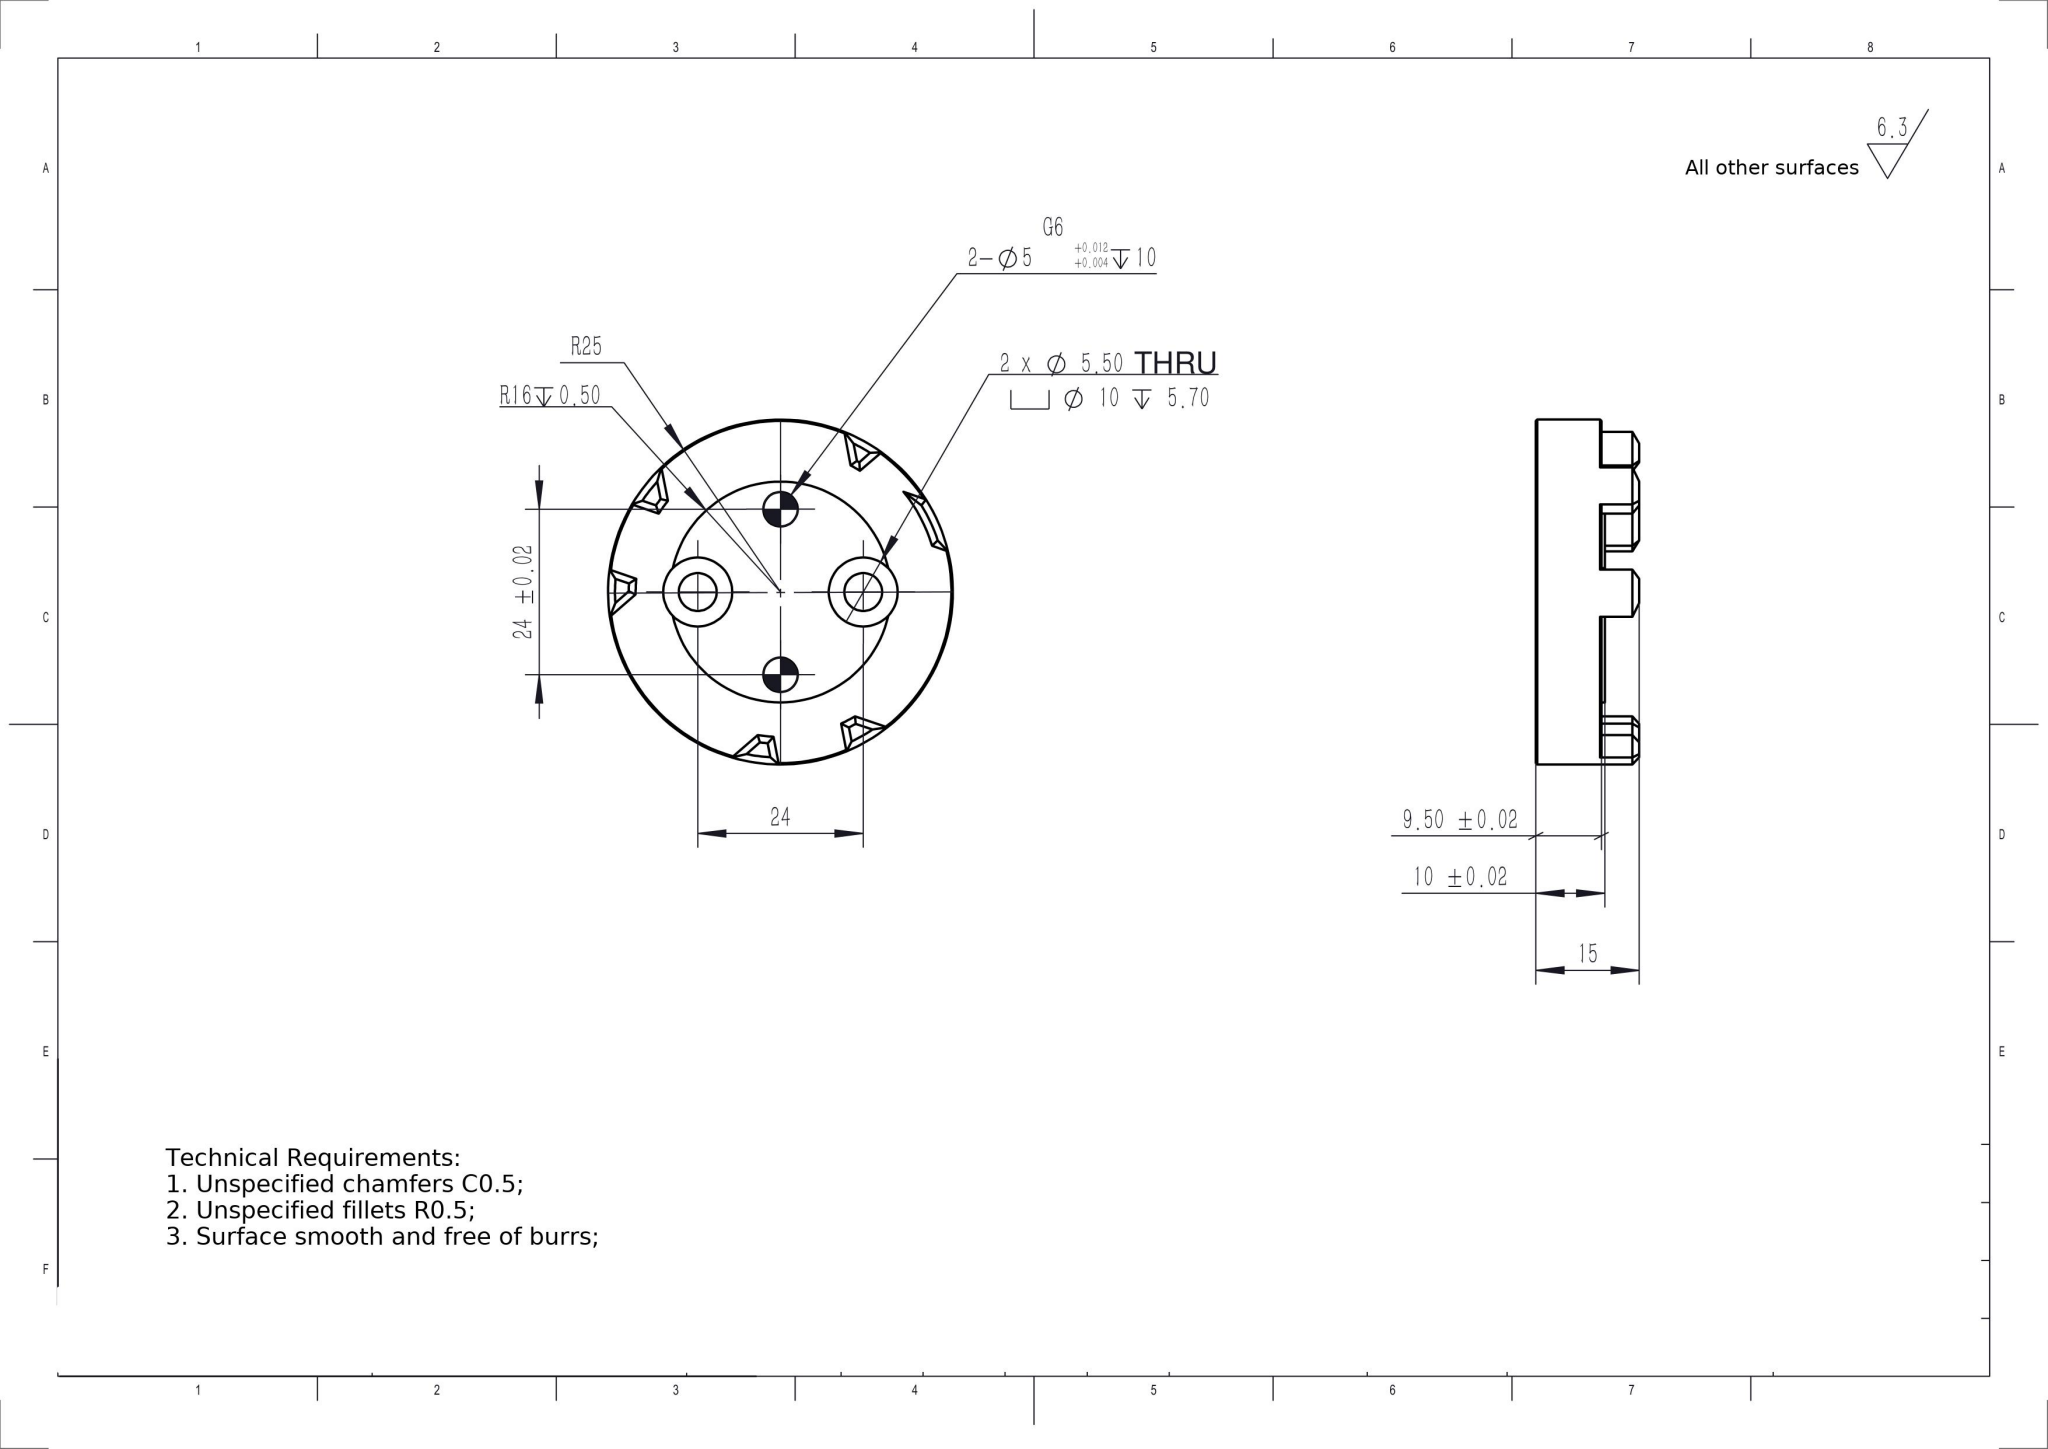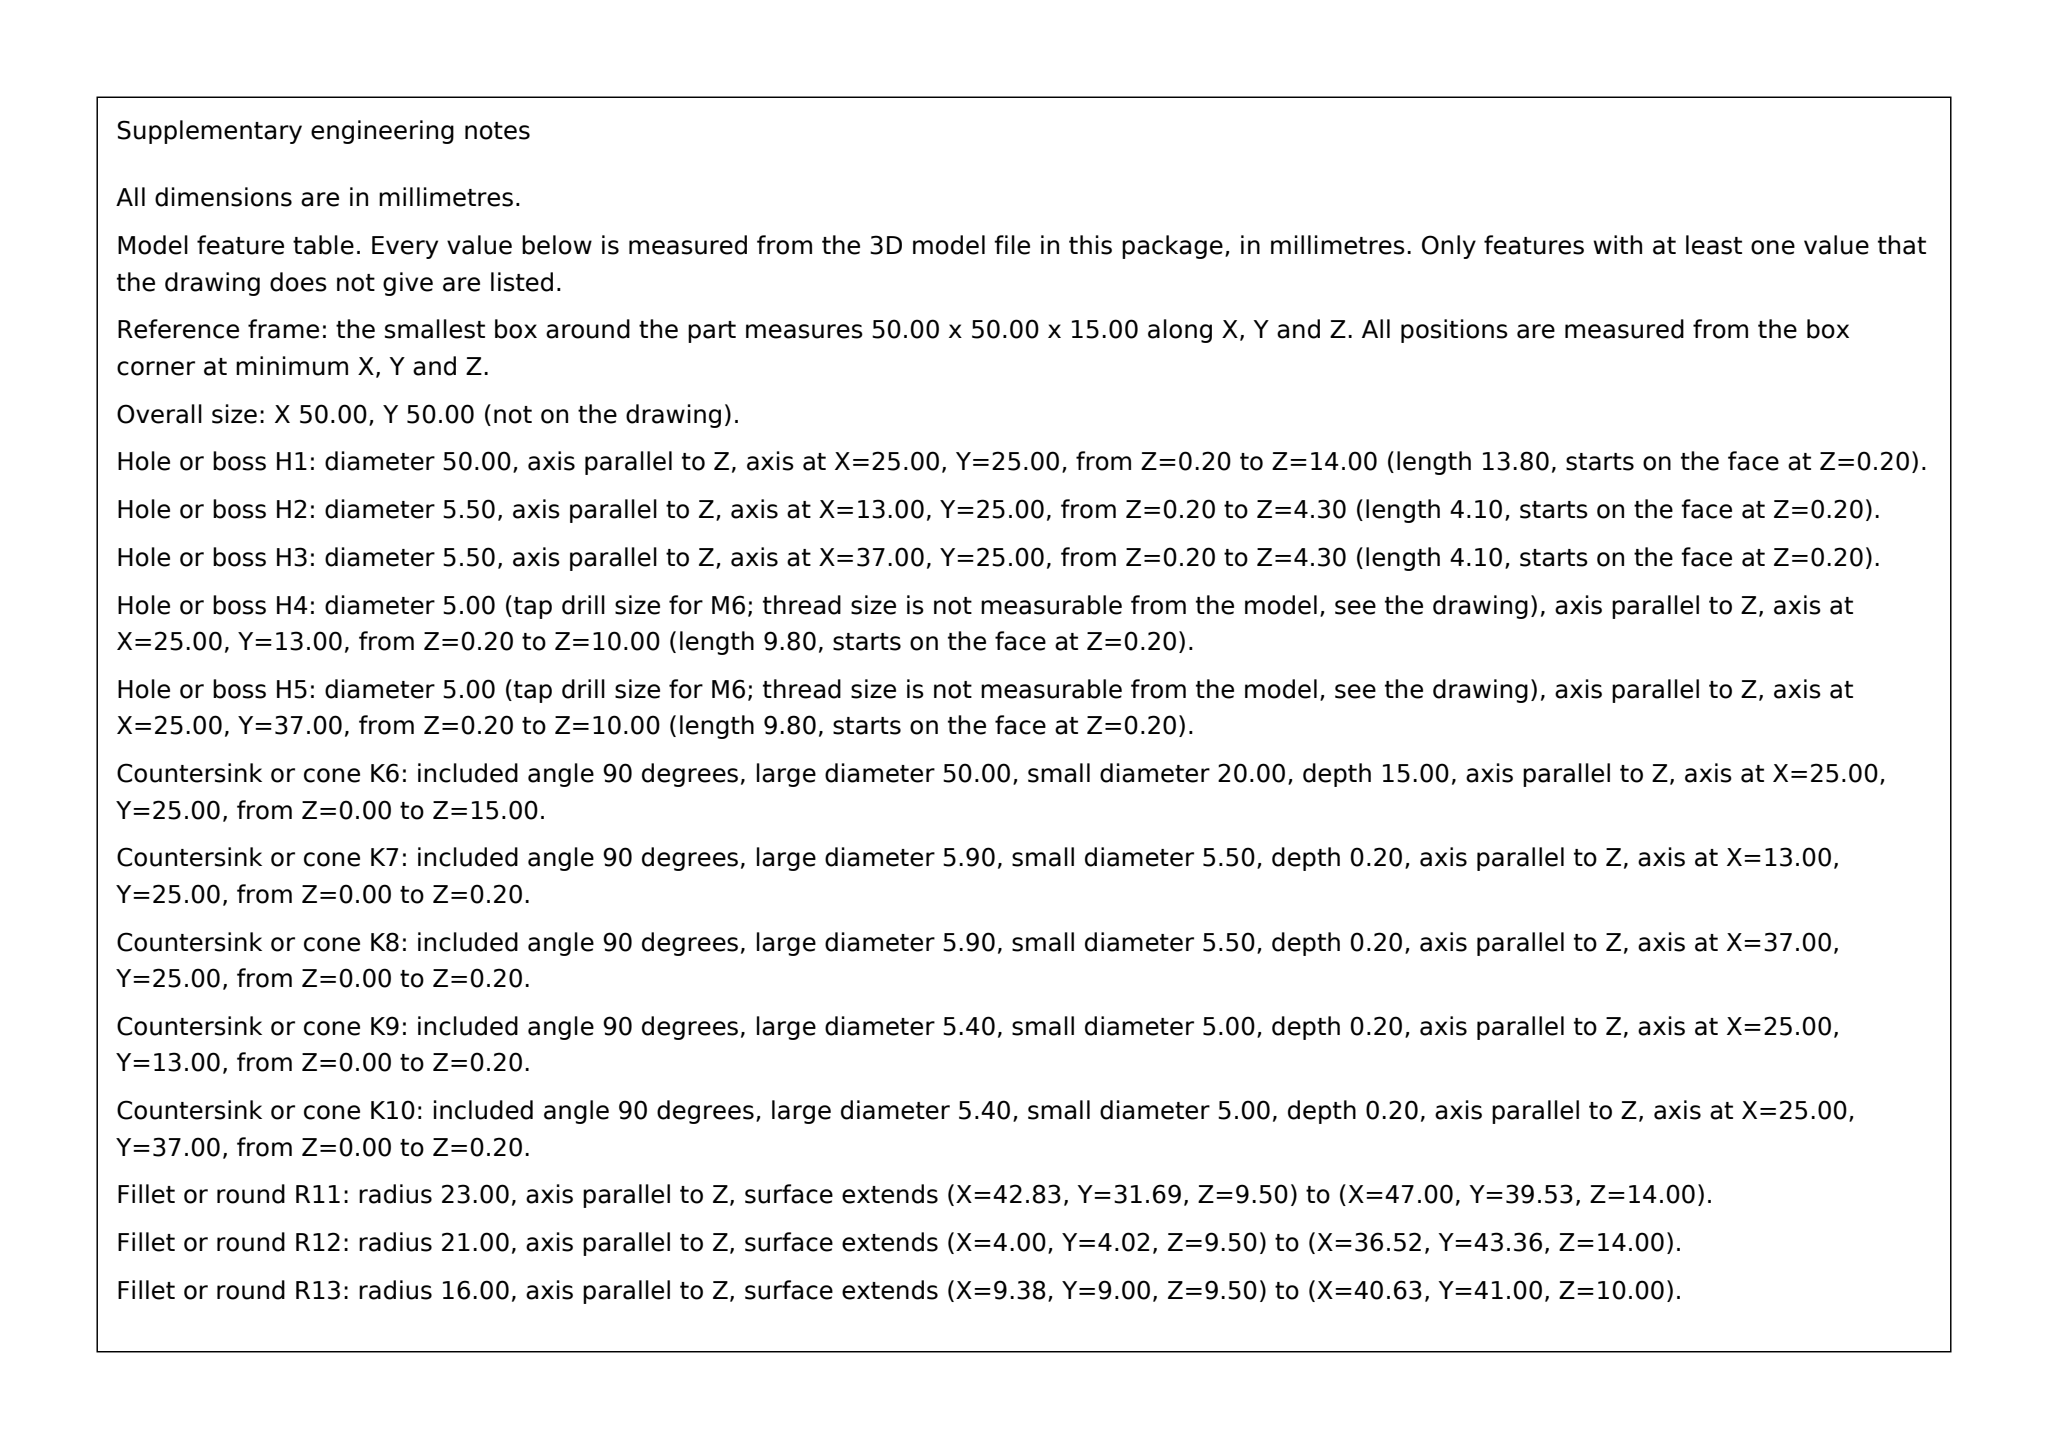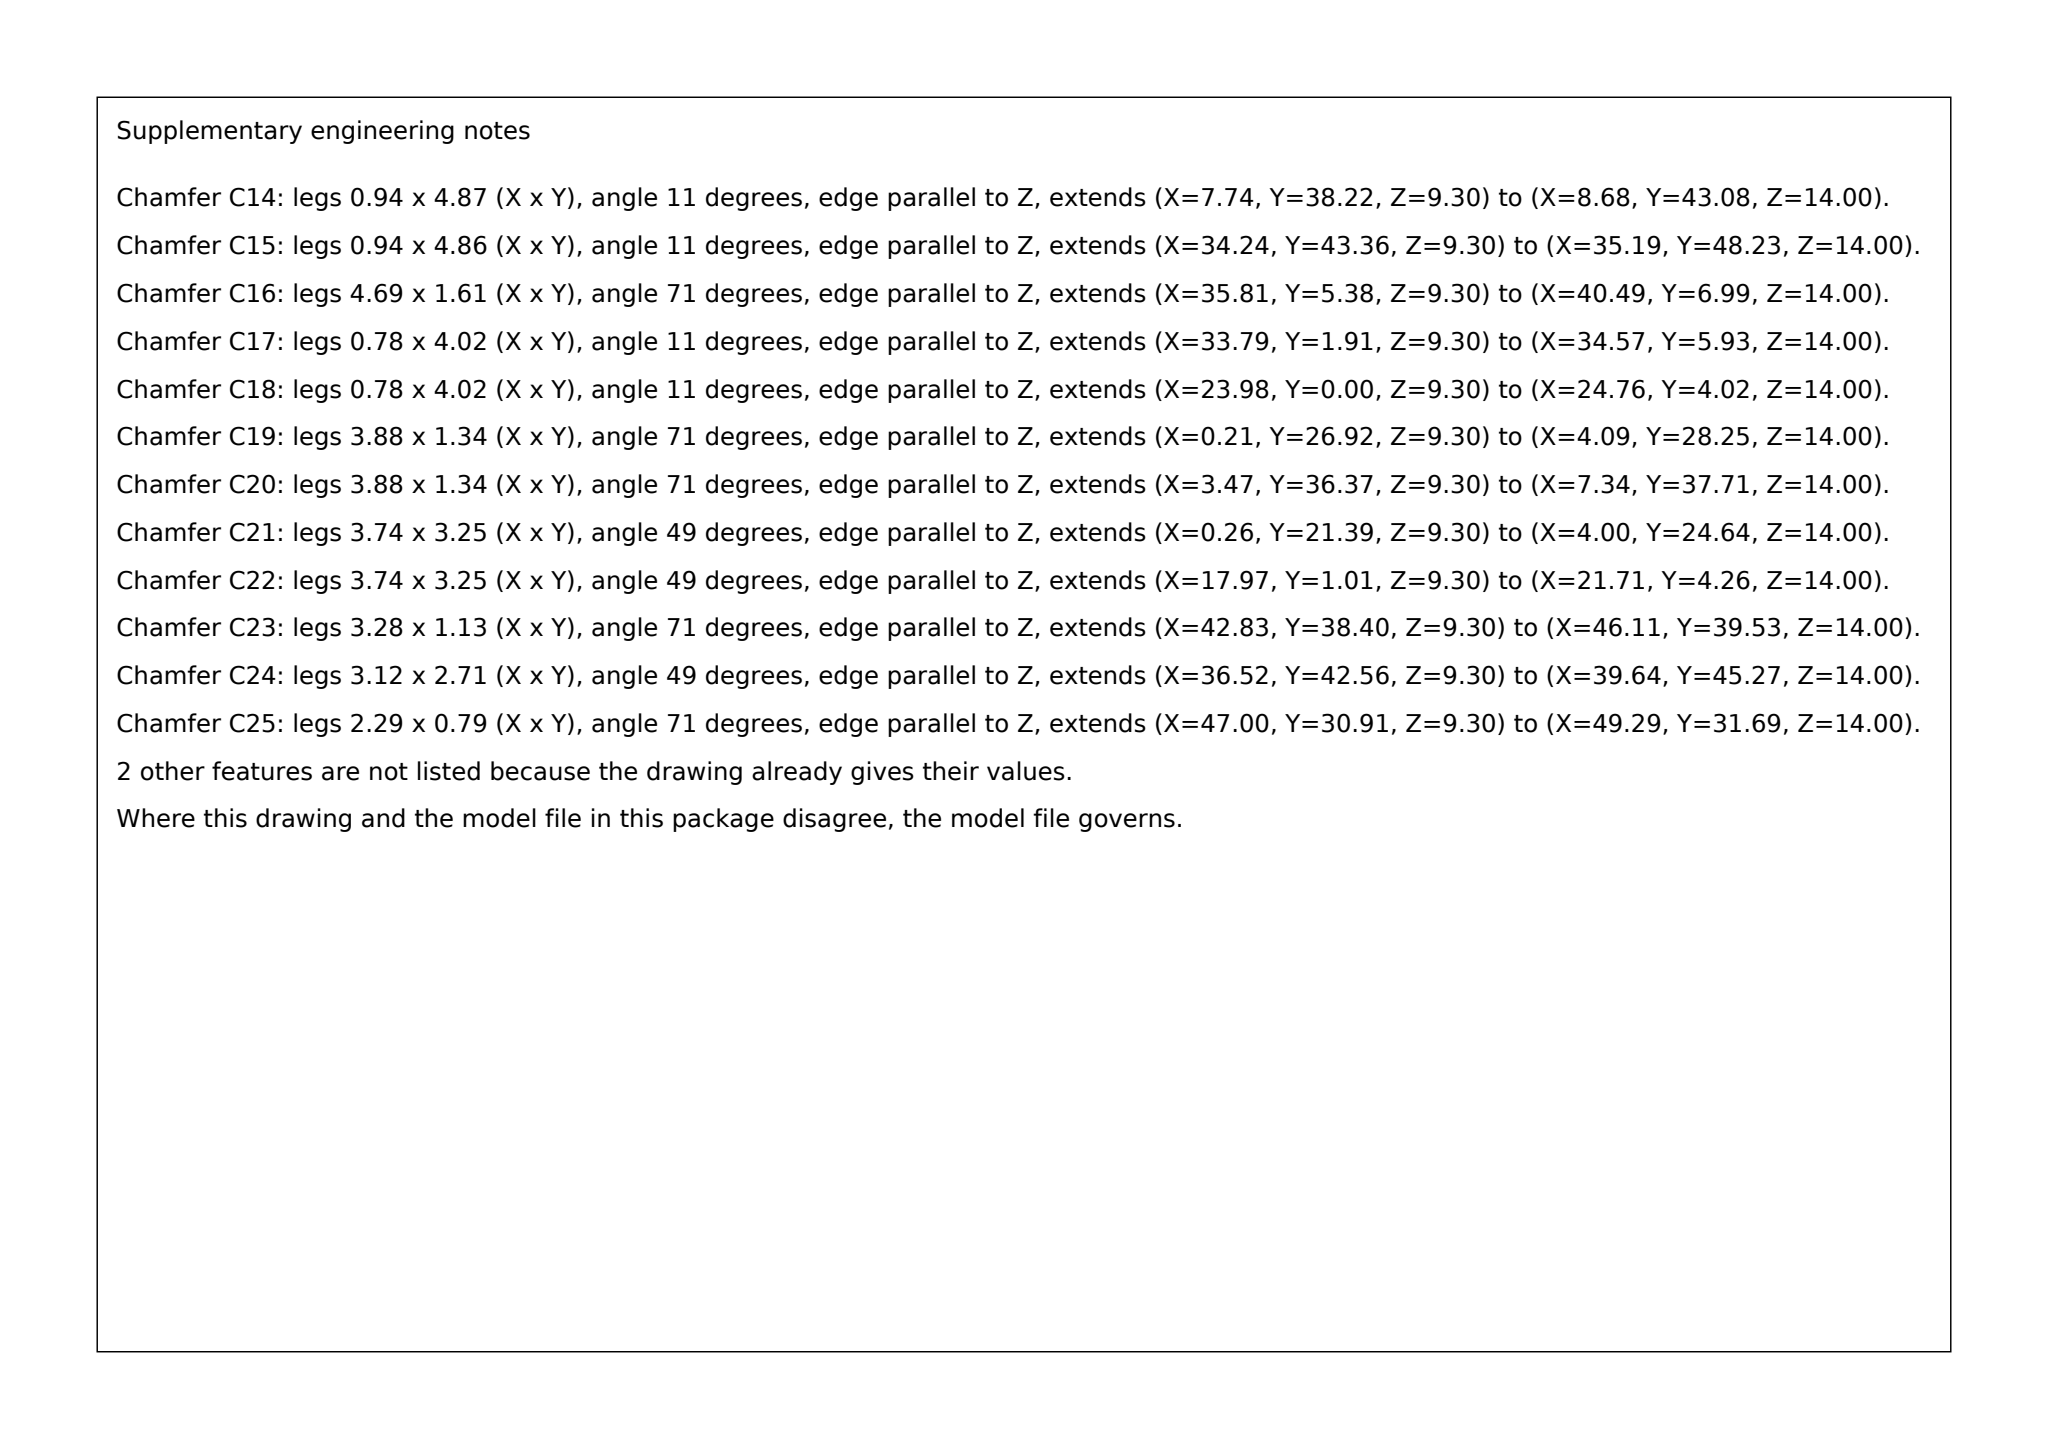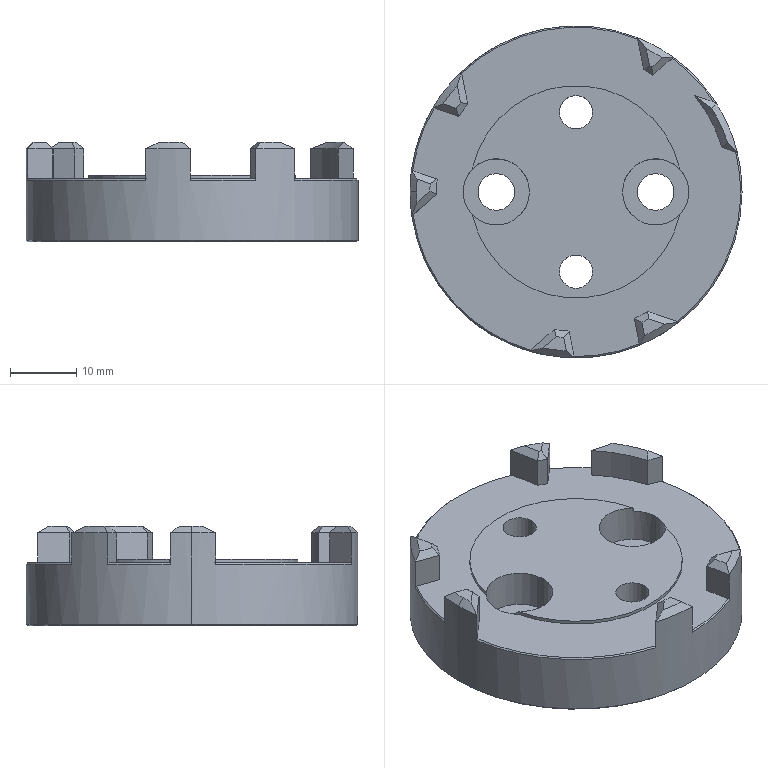Part | SolidWorks | mm | 1 solid | 85 faces | box 50 x 50 x 15 mm | volume 18098 mm3 | plane 34 | cone 29 | cylinder 22 | commonest cylinder face diameters 42 x5 5.5 x4 5 x4 10 x4 50 x2 32 x2 46 x1